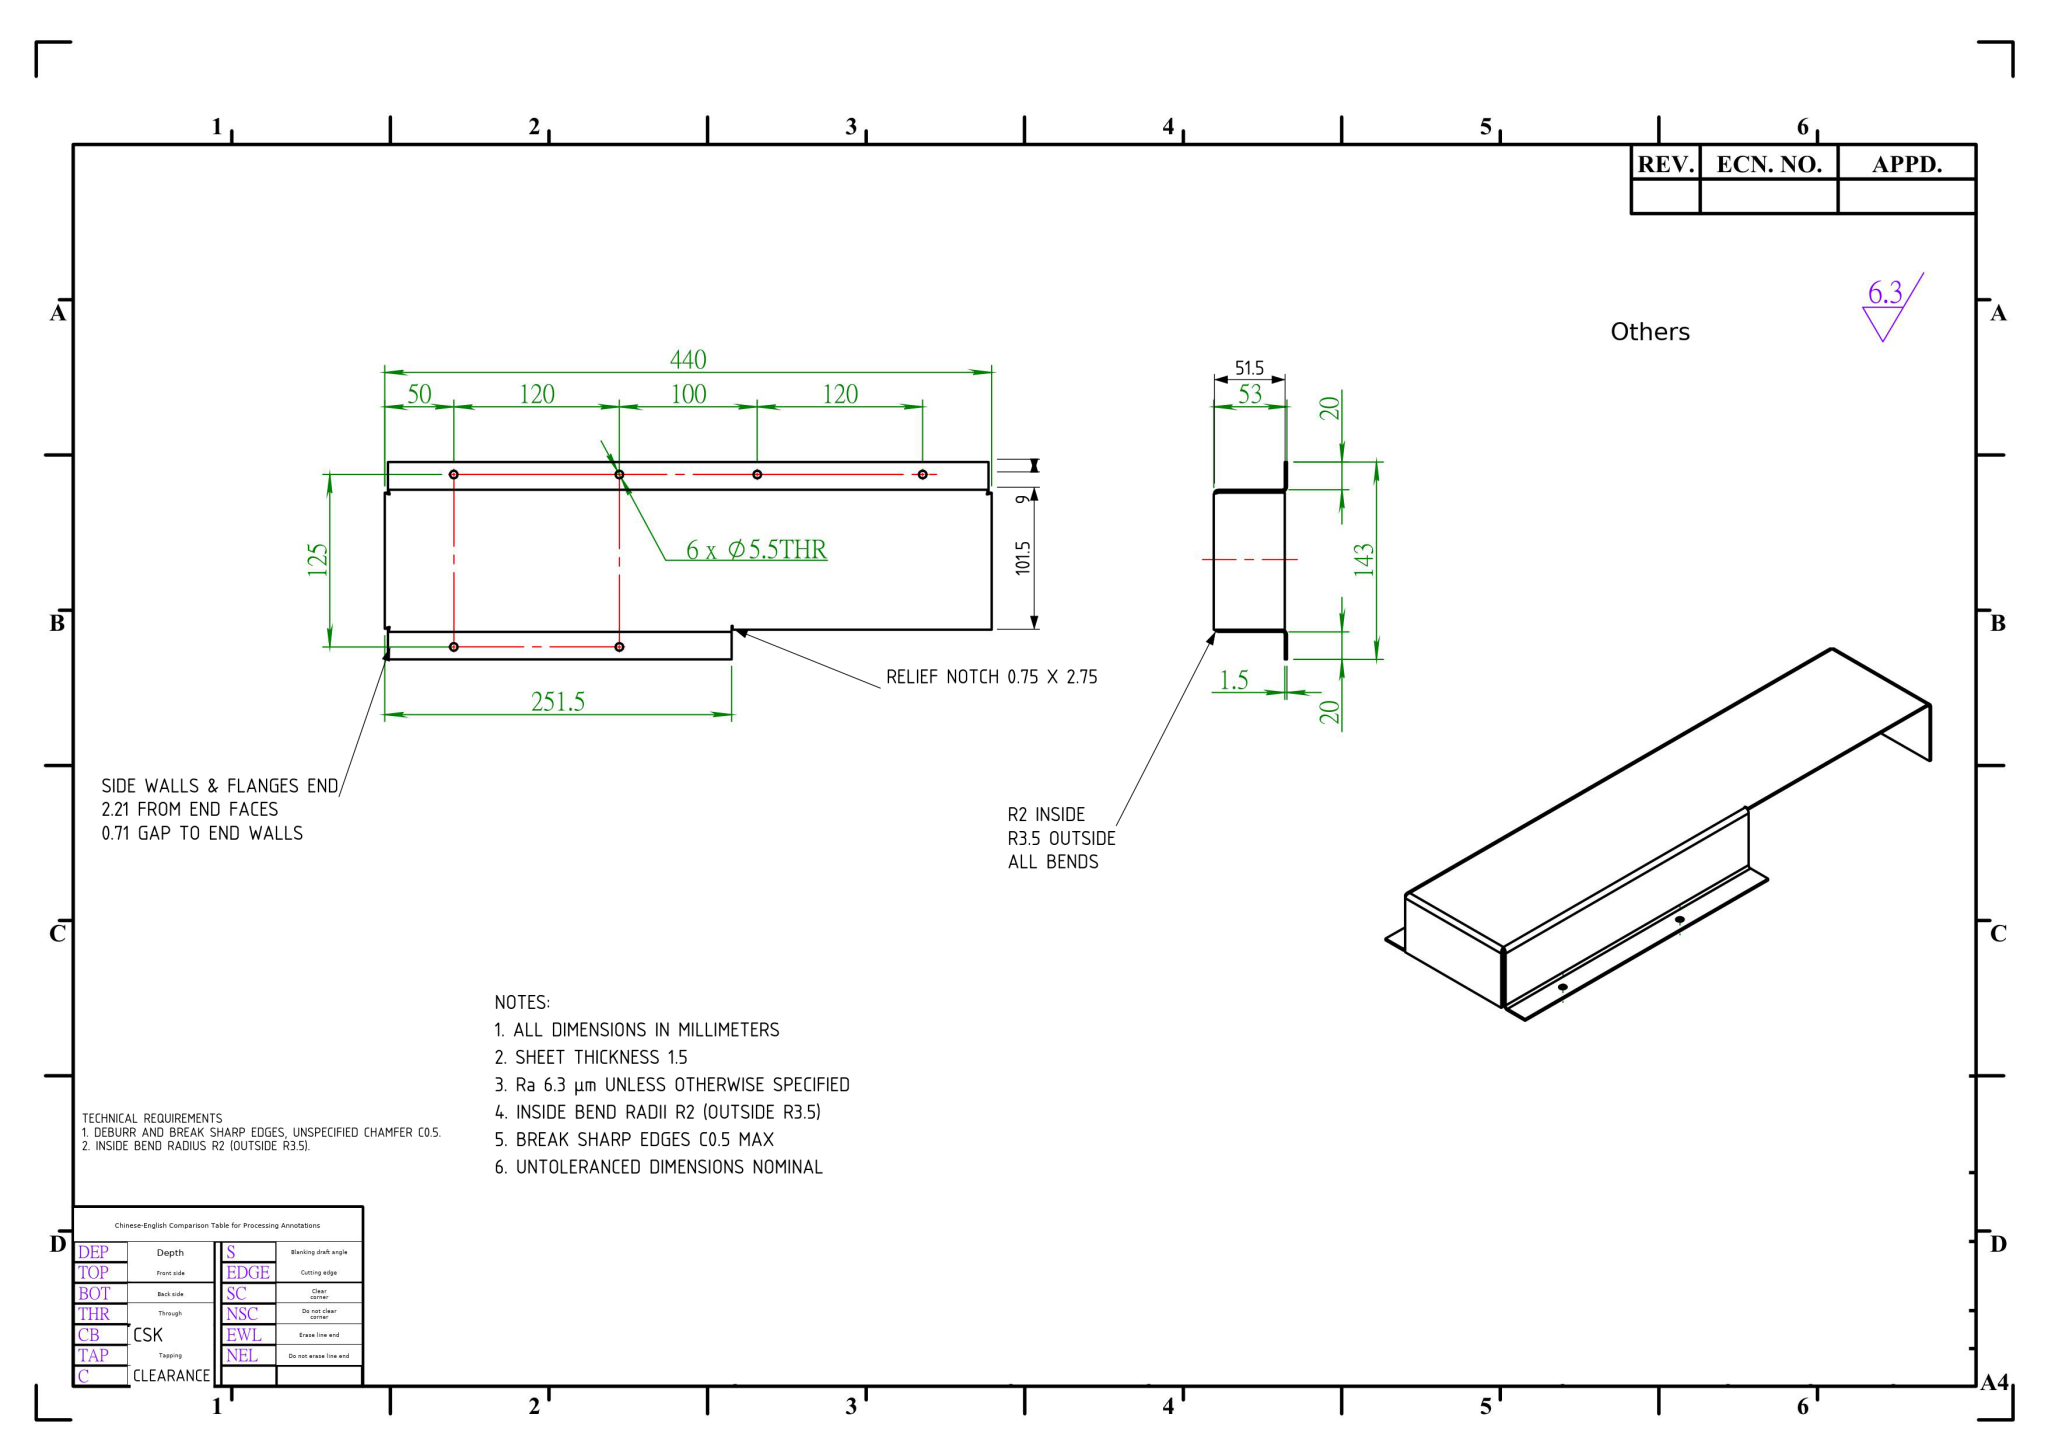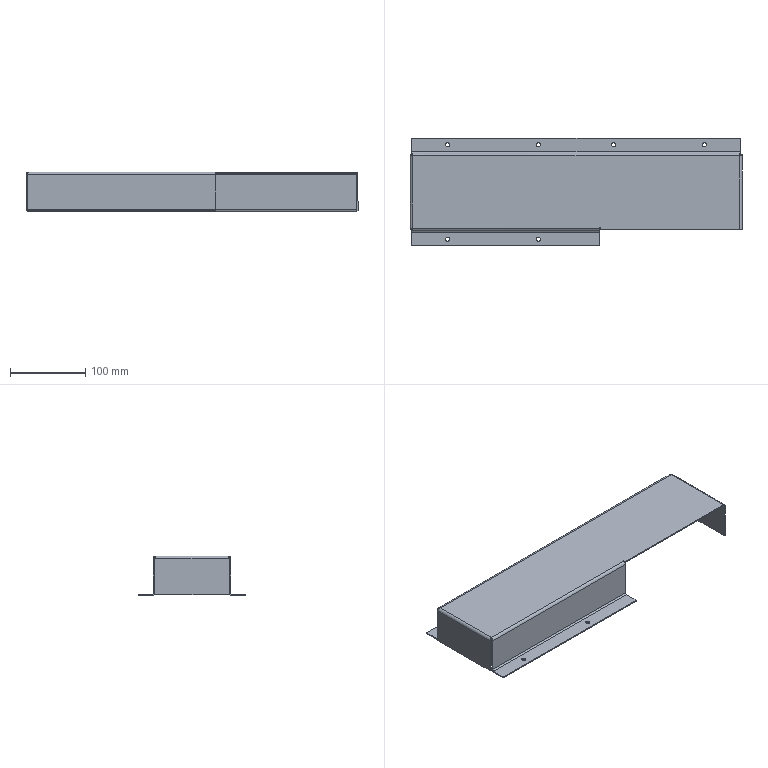Part | NX | mm | 1 solid | 70 faces | box 440 x 143 x 53 mm | volume 152818 mm3 | plane 40 | cylinder 24 | spline 6 | commonest cylinder face diameters 5.5 x12 7 x6 4 x6